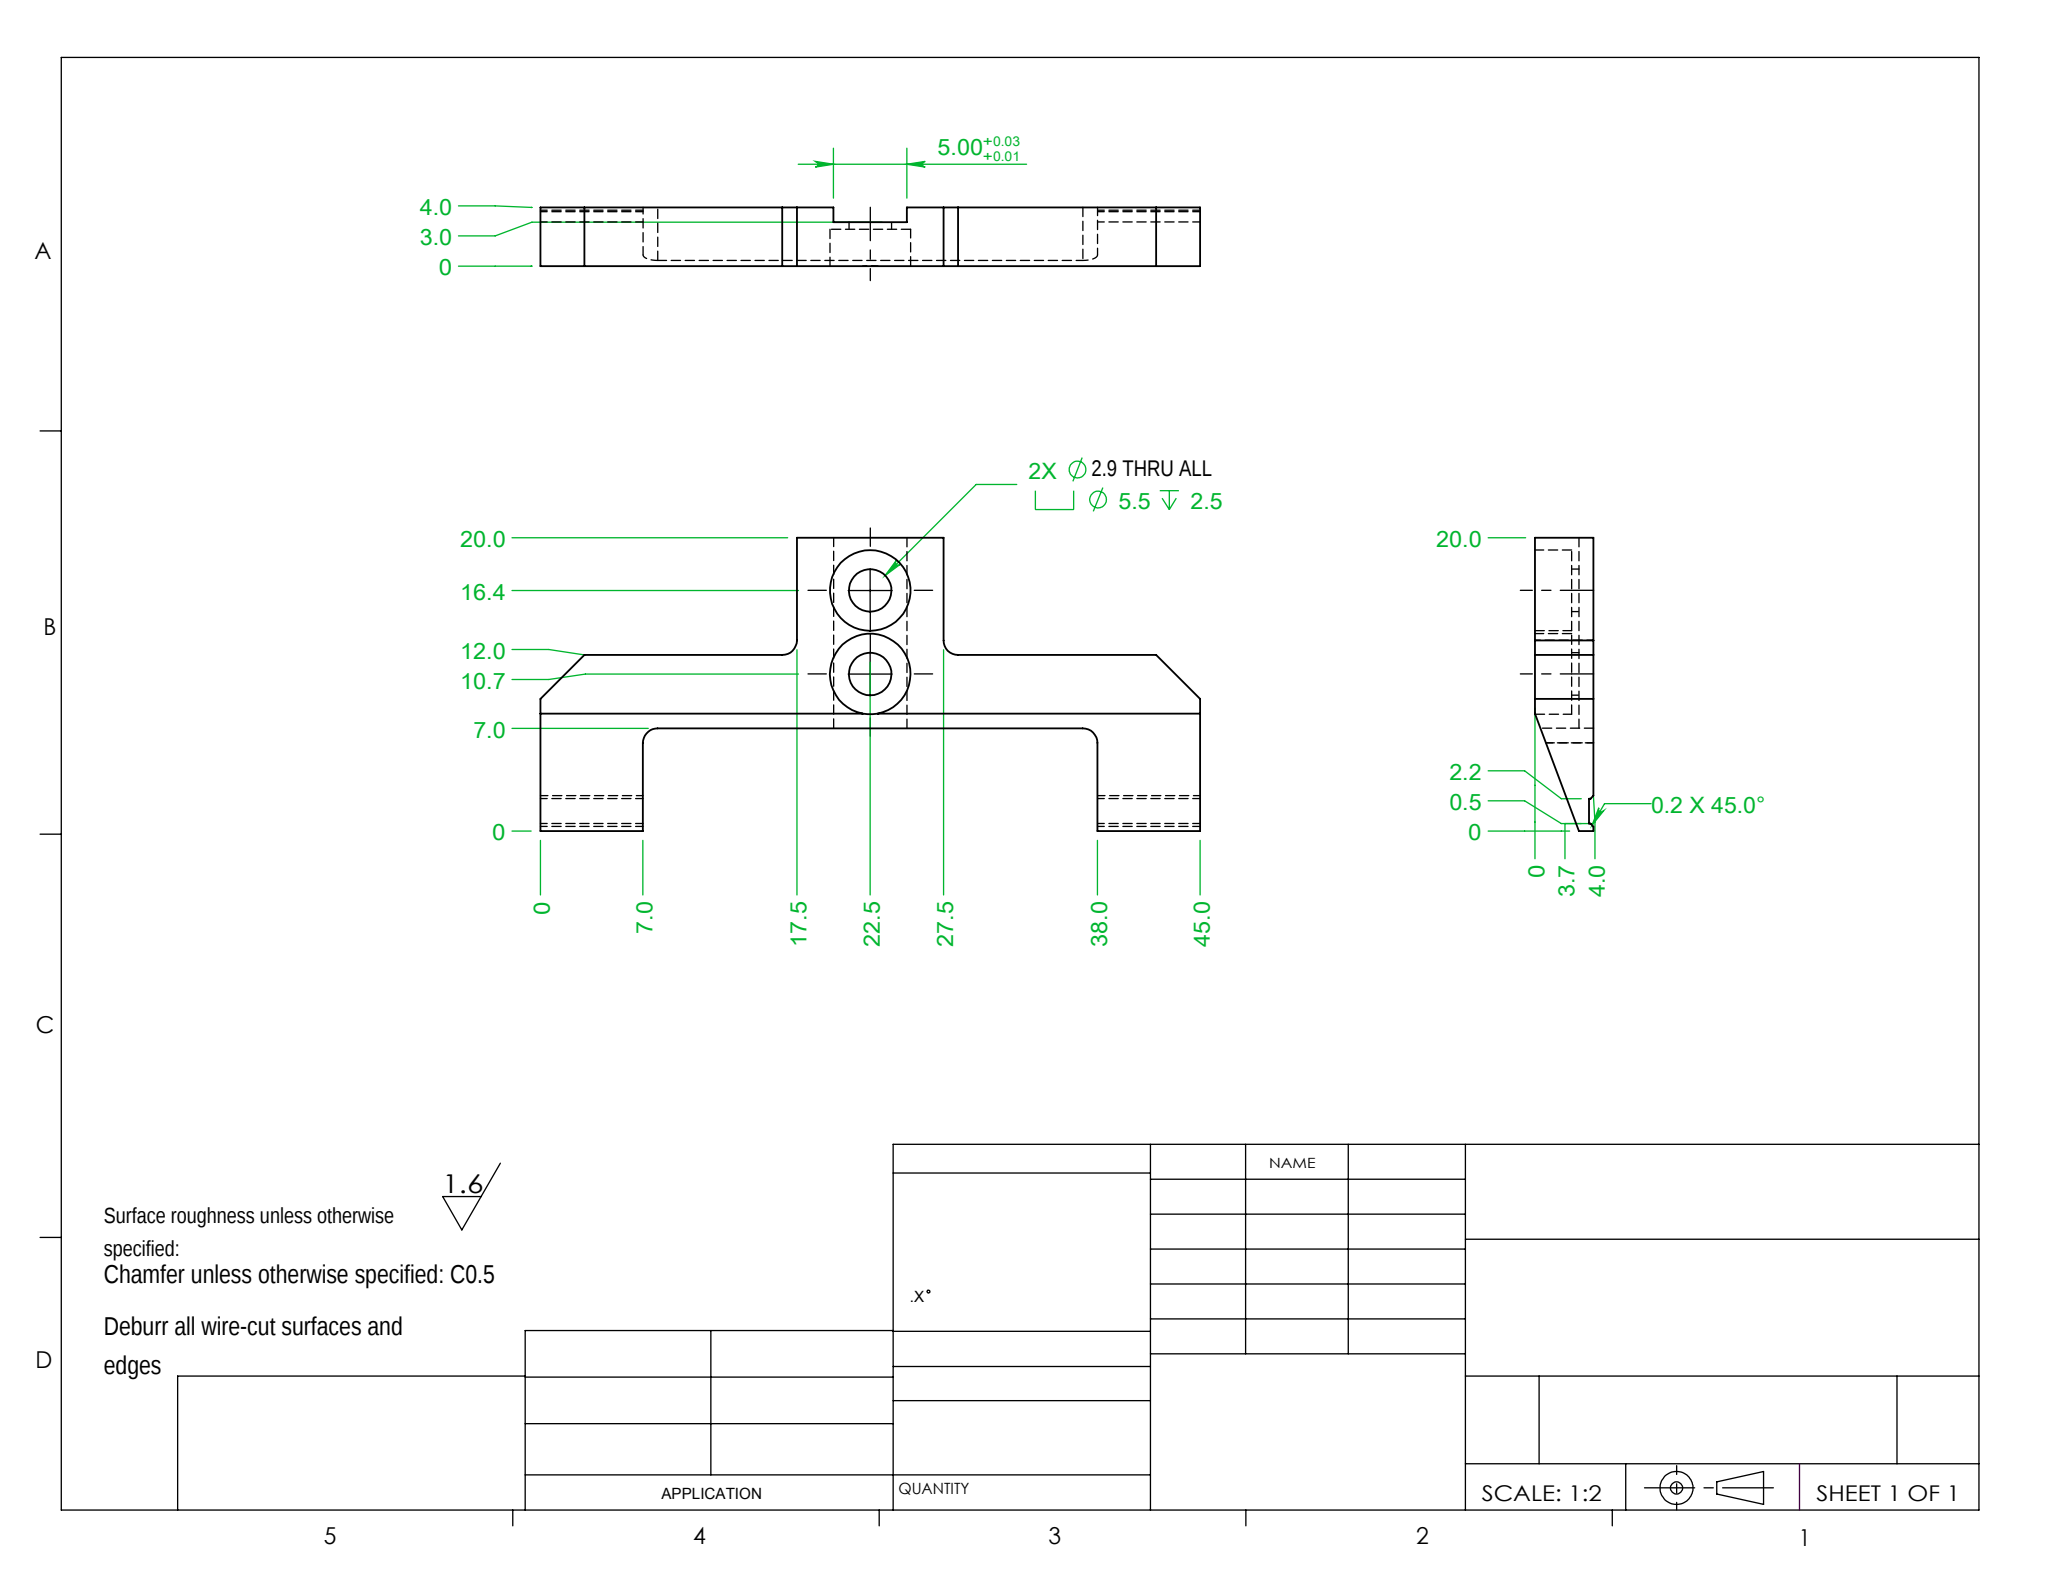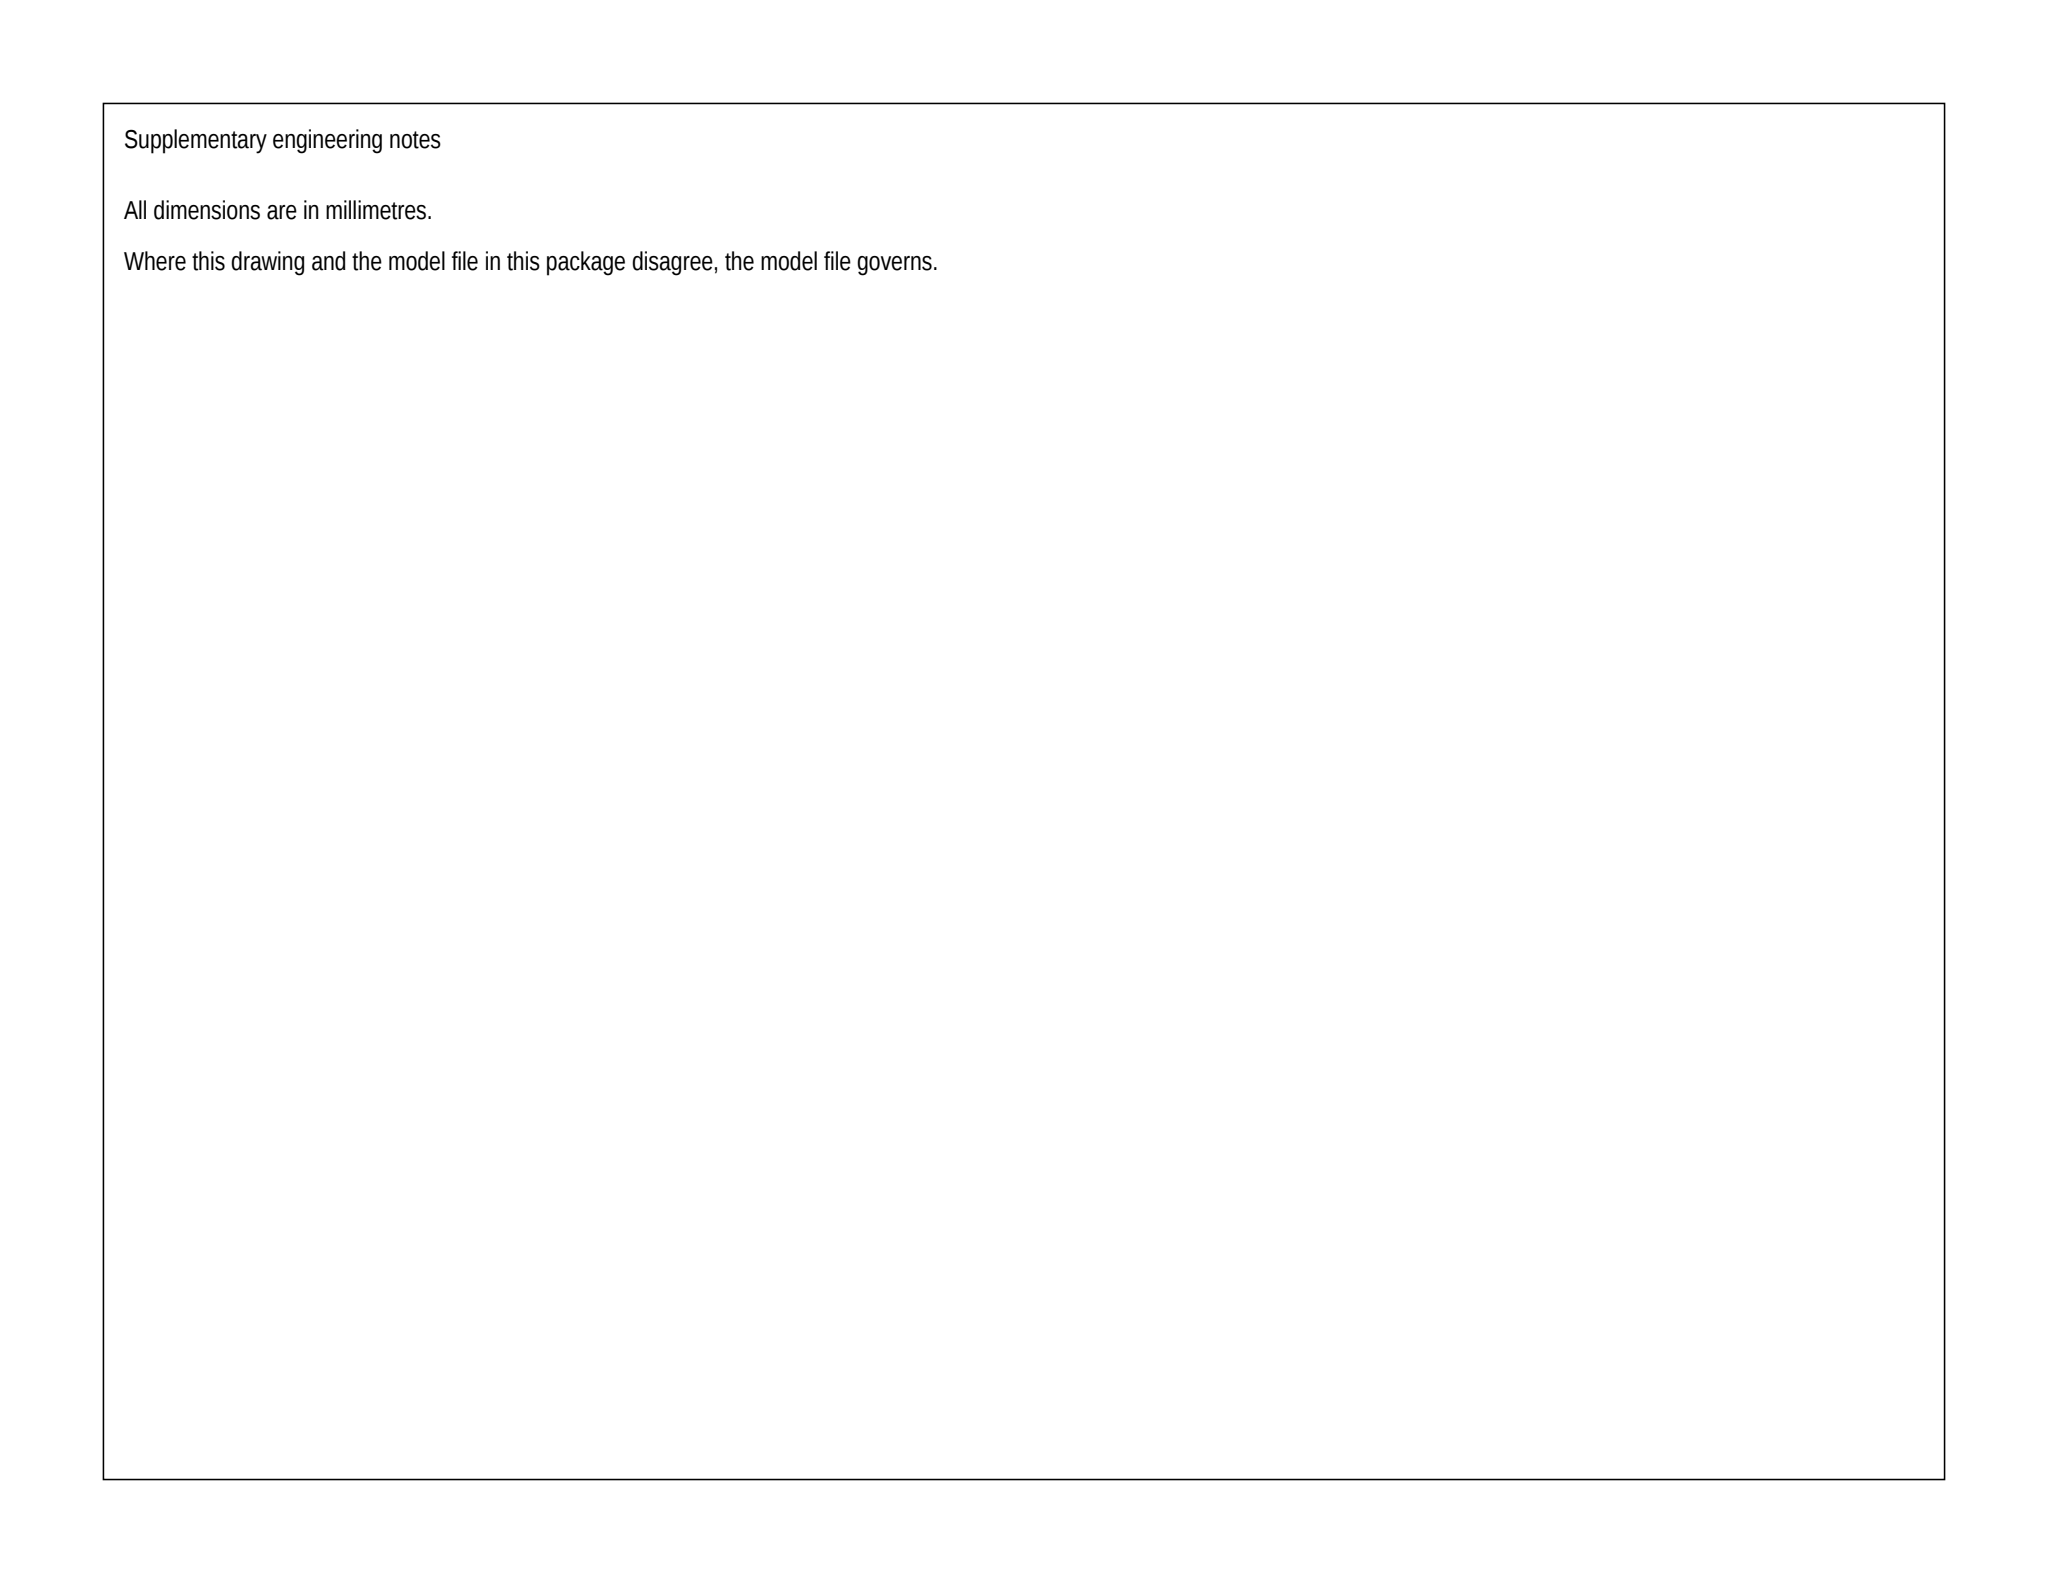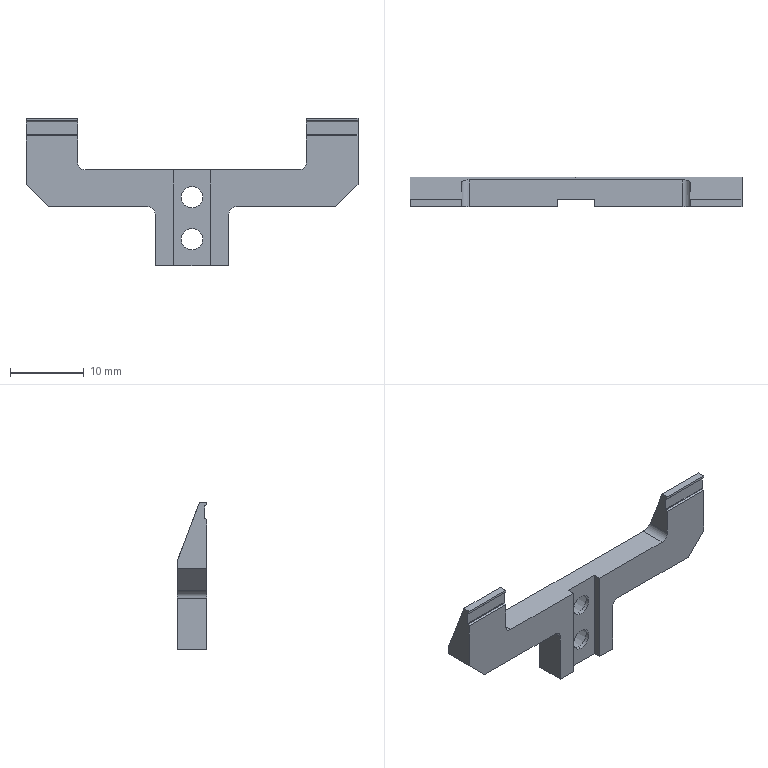Part | SolidWorks | mm | 1 solid | 47 faces | box 45 x 4 x 20 mm | volume 1207 mm3 | plane 35 | cylinder 12 | commonest cylinder face diameters 5.5 x4 2.9 x4 2 x4
build123d program:
from build123d import *

# Parameters (mm, degrees)
SKETCH1_W                                         = 45
SKETCH1_H                                         = 20
BOSS_EXTRUDE1_DEPTH                               = 4
SKETCH2_W                                         = 31
SKETCH2_H                                         = 7
CUT_EXTRUDE1_DEPTH                                = 50.406
SKETCH3_W                                         = 17.5
SKETCH3_H                                         = 8
CUT_EXTRUDE2_DEPTH                                = 50.406
SKETCH4_W                                         = 5
SKETCH4_H                                         = 13
CUT_EXTRUDE3_DEPTH                                = 1
FILLET1_R                                         = 1
CHAMFER1_SIZE                                     = 3
M2_5_HEX_SOCKET_HEAD_CAP_SCREW_CBORE1_D           = 2.9
M2_5_HEX_SOCKET_HEAD_CAP_SCREW_CBORE1_CBORE_D     = 5.5
M2_5_HEX_SOCKET_HEAD_CAP_SCREW_CBORE1_CBORE_DEPTH = 2.5
CUT_EXTRUDE4_DEPTH                                = 50.406
SKETCH8_W                                         = 1.7
SKETCH8_H                                         = 0.3
CUT_EXTRUDE5_DEPTH                                = 50.406
CHAMFER2_SIZE                                     = 0.2


with BuildPart() as part:
    # Sketch1 → Boss-Extrude1 (new body)
    with BuildSketch(Plane(origin=(0, 0, 0), x_dir=(1, 0, 0), z_dir=(0, 1, 0))):
        with Locations((22.5, 10)):
            Rectangle(SKETCH1_W, SKETCH1_H)
    extrude(amount=BOSS_EXTRUDE1_DEPTH)

    # Sketch2 → Cut-Extrude1 (cut, through all)
    with BuildSketch(Plane(origin=(0, 4, 0), x_dir=(1, 0, 0), z_dir=(0, 1, 0))):
        with Locations((22.5, 3.5)):
            Rectangle(SKETCH2_W, SKETCH2_H)
    extrude(amount=-CUT_EXTRUDE1_DEPTH, mode=Mode.SUBTRACT)

    # Sketch3 → Cut-Extrude2 (cut, through all)
    with BuildSketch(Plane(origin=(0, 4, 0), x_dir=(1, 0, 0), z_dir=(0, 1, 0))):
        with Locations((36.25, 16)):
            Rectangle(SKETCH3_W, SKETCH3_H)
        with Locations((8.75, 16)):
            Rectangle(SKETCH3_W, SKETCH3_H)
    extrude(amount=-CUT_EXTRUDE2_DEPTH, mode=Mode.SUBTRACT)

    # Sketch4 → Cut-Extrude3 (cut)
    with BuildSketch(Plane.XZ):
        with Locations((22.5, -13.5)):
            Rectangle(SKETCH4_W, SKETCH4_H)
    extrude(amount=-CUT_EXTRUDE3_DEPTH, mode=Mode.SUBTRACT)

    # Fillet1
    fillet1_edges = [part.edges().sort_by_distance(p)[0] for p in [
        (7, 2, -7),
        (38, 2, -7),
        (27.5, 2, -12),
        (17.5, 2, -12),
    ]]
    fillet(fillet1_edges, radius=FILLET1_R)

    # Chamfer1
    chamfer1_edges = [part.edges().sort_by_distance(p)[0] for p in [
        (45, 2, -12),
        (0, 2, -12),
    ]]
    chamfer(chamfer1_edges, length=CHAMFER1_SIZE)

    # M2.5 Hex Socket Head Cap Screw CBORE1 (through all)
    with Locations(Plane(origin=(0, 4, 0), x_dir=(1, 0, 0), z_dir=(0, 1, 0))):
        with Locations((22.5, 16.4), (22.5, 10.7)):
            CounterBoreHole(M2_5_HEX_SOCKET_HEAD_CAP_SCREW_CBORE1_D / 2, M2_5_HEX_SOCKET_HEAD_CAP_SCREW_CBORE1_CBORE_D / 2, M2_5_HEX_SOCKET_HEAD_CAP_SCREW_CBORE1_CBORE_DEPTH)

    # Sketch7 → Cut-Extrude4 (cut, through all)
    with BuildSketch(Plane(origin=(45, 0, 0), x_dir=(0, 0, -1), z_dir=(1, 0, 0))):
        Polygon((0, 4), (8, 4), (0, 1), align=None)
    extrude(amount=-CUT_EXTRUDE4_DEPTH, mode=Mode.SUBTRACT)

    # Sketch8 → Cut-Extrude5 (cut, through all)
    with BuildSketch(Plane(origin=(45, 0, 0), x_dir=(0, 0, -1), z_dir=(1, 0, 0))):
        with Locations((1.35, 0.15)):
            Rectangle(SKETCH8_W, SKETCH8_H)
    extrude(amount=-CUT_EXTRUDE5_DEPTH, mode=Mode.SUBTRACT)

    # Chamfer2
    chamfer2_edges = [part.edges().sort_by_distance(p)[0] for p in [
        (3.5, 0, -2.2),
        (41.5, 0, -2.2),
        (3.5, 0, -0.5),
        (41.5, 0, -0.5),
    ]]
    chamfer(chamfer2_edges, length=CHAMFER2_SIZE)


solid = part.part